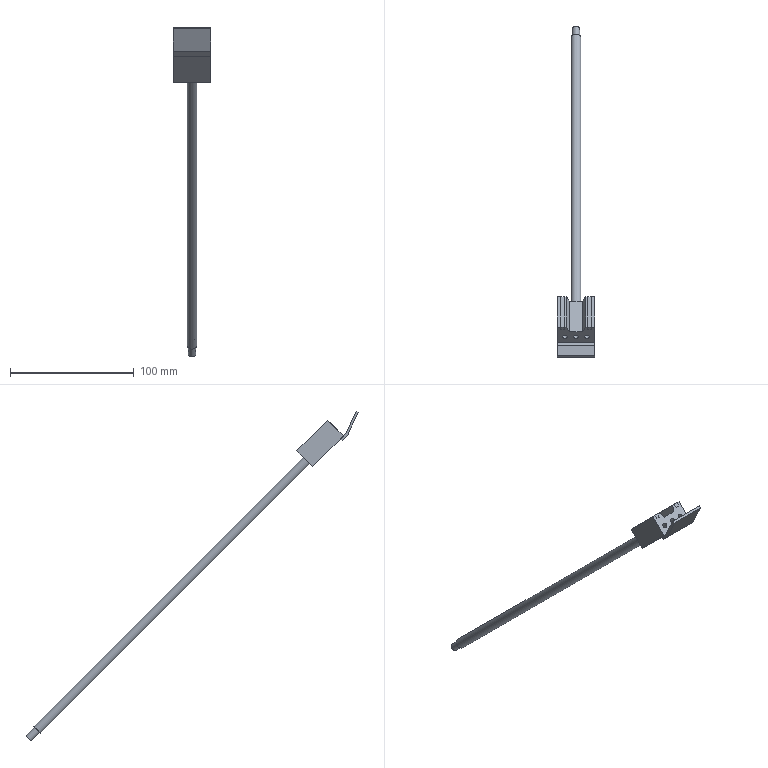Component | NX | MODEL1 | 4 solids | 51 faces | volume 23884 mm3 | plane 44 | cylinder 7 | commonest cylinder face diameters 4 x4 6 x2 8 x1